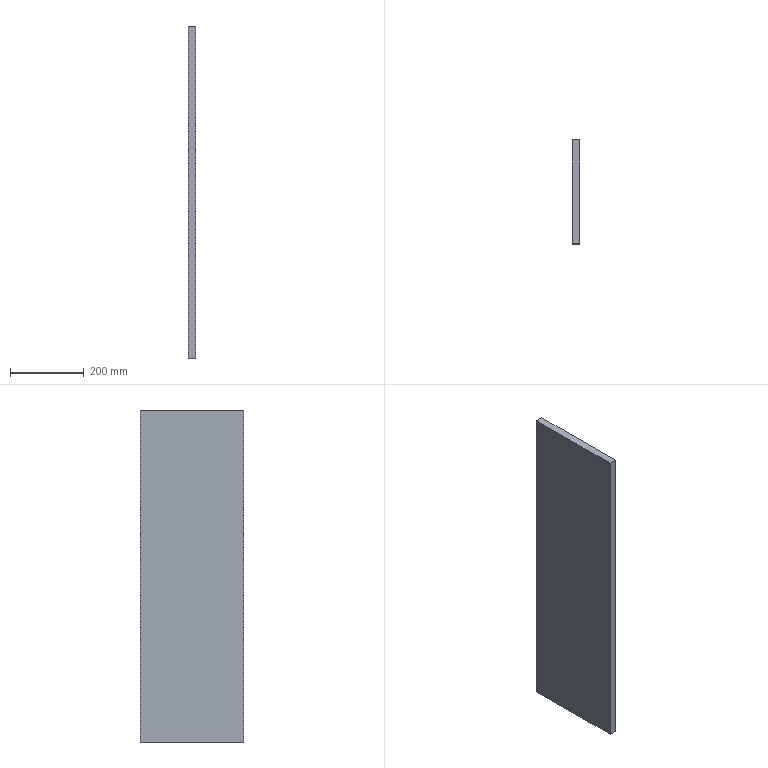Component | SolidWorks | BasePlate-1 | 1 solid | 6 faces | box 20 x 281.2 x 900 mm | volume 5061600 mm3 | plane 6 | material 45
build123d program:
from build123d import *

# Parameters (mm, degrees)
SKETCH1_W           = 900
SKETCH1_H           = 281.2
BOSS_EXTRUDE1_DEPTH = 20


with BuildPart() as part:
    # Sketch1 → Boss-Extrude1 (new body)
    with BuildSketch(Plane.XY):
        Rectangle(SKETCH1_W, SKETCH1_H)
    extrude(amount=BOSS_EXTRUDE1_DEPTH)


solid = part.part

# Placed as in the assembly
solid = solid.moved(Location((-261.359, -192.885, 1152), (0, 90, 0)))
STEP:
#1=CARTESIAN_POINT('',(-9.502,-2.058,27.638));
#2=VERTEX_POINT('',#1);
#3=CARTESIAN_POINT('',(-9.502,-13.129,27.638));
#4=VERTEX_POINT('',#3);
#5=CARTESIAN_POINT('',(-9.502,-13.129,27.638));
#6=DIRECTION('',(0.,-1.,0.));
#7=VECTOR('',#6,39.37);
#8=LINE('',#5,#7);
#9=EDGE_CURVE('',#2,#4,#8,.T.);
#10=ORIENTED_EDGE('',*,*,#9,.T.);
#11=CARTESIAN_POINT('',(-10.29,-13.129,27.638));
#12=VERTEX_POINT('',#11);
#13=CARTESIAN_POINT('',(-10.29,-13.129,27.638));
#14=DIRECTION('',(1.,0.,0.));
#15=VECTOR('',#14,39.37);
#16=LINE('',#13,#15);
#17=EDGE_CURVE('',#12,#4,#16,.T.);
#18=ORIENTED_EDGE('',*,*,#17,.F.);
#19=CARTESIAN_POINT('',(-10.29,-2.058,27.638));
#20=VERTEX_POINT('',#19);
#21=CARTESIAN_POINT('',(-10.29,-13.129,27.638));
#22=DIRECTION('',(0.,-1.,0.));
#23=VECTOR('',#22,39.37);
#24=LINE('',#21,#23);
#25=EDGE_CURVE('',#20,#12,#24,.T.);
#26=ORIENTED_EDGE('',*,*,#25,.F.);
#27=CARTESIAN_POINT('',(-10.29,-2.058,27.638));
#28=DIRECTION('',(1.,0.,0.));
#29=VECTOR('',#28,39.37);
#30=LINE('',#27,#29);
#31=EDGE_CURVE('',#20,#2,#30,.T.);
#32=ORIENTED_EDGE('',*,*,#31,.T.);
#33=EDGE_LOOP('',(#10,#18,#26,#32));
#34=FACE_OUTER_BOUND('',#33,.T.);
#35=CARTESIAN_POINT('',(-10.29,-13.129,27.638));
#36=DIRECTION('',(0.,0.,1.));
#37=DIRECTION('',(1.,0.,0.));
#38=AXIS2_PLACEMENT_3D('',#35,#36,#37);
#39=PLANE('',#38);
#40=ADVANCED_FACE('',(#34),#39,.F.);
#41=CARTESIAN_POINT('',(-9.502,-13.129,63.071));
#42=VERTEX_POINT('',#41);
#43=CARTESIAN_POINT('',(-9.502,-13.129,63.071));
#44=DIRECTION('',(0.,0.,1.));
#45=VECTOR('',#44,39.37);
#46=LINE('',#43,#45);
#47=EDGE_CURVE('',#4,#42,#46,.T.);
#48=ORIENTED_EDGE('',*,*,#47,.T.);
#49=CARTESIAN_POINT('',(-10.29,-13.129,63.071));
#50=VERTEX_POINT('',#49);
#51=CARTESIAN_POINT('',(-10.29,-13.129,63.071));
#52=DIRECTION('',(1.,0.,0.));
#53=VECTOR('',#52,39.37);
#54=LINE('',#51,#53);
#55=EDGE_CURVE('',#50,#42,#54,.T.);
#56=ORIENTED_EDGE('',*,*,#55,.F.);
#57=CARTESIAN_POINT('',(-10.29,-13.129,63.071));
#58=DIRECTION('',(0.,0.,1.));
#59=VECTOR('',#58,39.37);
#60=LINE('',#57,#59);
#61=EDGE_CURVE('',#12,#50,#60,.T.);
#62=ORIENTED_EDGE('',*,*,#61,.F.);
#63=ORIENTED_EDGE('',*,*,#17,.T.);
#64=EDGE_LOOP('',(#48,#56,#62,#63));
#65=FACE_OUTER_BOUND('',#64,.T.);
#66=CARTESIAN_POINT('',(-10.29,-13.129,63.071));
#67=DIRECTION('',(0.,1.,-0.));
#68=DIRECTION('',(0.,-0.,-1.));
#69=AXIS2_PLACEMENT_3D('',#66,#67,#68);
#70=PLANE('',#69);
#71=ADVANCED_FACE('',(#65),#70,.F.);
#72=CARTESIAN_POINT('',(-9.502,-2.058,63.071));
#73=VERTEX_POINT('',#72);
#74=CARTESIAN_POINT('',(-9.502,-13.129,63.071));
#75=DIRECTION('',(0.,1.,0.));
#76=VECTOR('',#75,39.37);
#77=LINE('',#74,#76);
#78=EDGE_CURVE('',#42,#73,#77,.T.);
#79=ORIENTED_EDGE('',*,*,#78,.T.);
#80=CARTESIAN_POINT('',(-10.29,-2.058,63.071));
#81=VERTEX_POINT('',#80);
#82=CARTESIAN_POINT('',(-10.29,-2.058,63.071));
#83=DIRECTION('',(1.,0.,0.));
#84=VECTOR('',#83,39.37);
#85=LINE('',#82,#84);
#86=EDGE_CURVE('',#81,#73,#85,.T.);
#87=ORIENTED_EDGE('',*,*,#86,.F.);
#88=CARTESIAN_POINT('',(-10.29,-13.129,63.071));
#89=DIRECTION('',(0.,1.,0.));
#90=VECTOR('',#89,39.37);
#91=LINE('',#88,#90);
#92=EDGE_CURVE('',#50,#81,#91,.T.);
#93=ORIENTED_EDGE('',*,*,#92,.F.);
#94=ORIENTED_EDGE('',*,*,#55,.T.);
#95=EDGE_LOOP('',(#79,#87,#93,#94));
#96=FACE_OUTER_BOUND('',#95,.T.);
#97=CARTESIAN_POINT('',(-10.29,-13.129,63.071));
#98=DIRECTION('',(0.,0.,-1.));
#99=DIRECTION('',(-1.,0.,0.));
#100=AXIS2_PLACEMENT_3D('',#97,#98,#99);
#101=PLANE('',#100);
#102=ADVANCED_FACE('',(#96),#101,.F.);
#103=CARTESIAN_POINT('',(-9.502,-2.058,63.071));
#104=DIRECTION('',(0.,-0.,-1.));
#105=VECTOR('',#104,39.37);
#106=LINE('',#103,#105);
#107=EDGE_CURVE('',#73,#2,#106,.T.);
#108=ORIENTED_EDGE('',*,*,#107,.T.);
#109=ORIENTED_EDGE('',*,*,#31,.F.);
#110=CARTESIAN_POINT('',(-10.29,-2.058,63.071));
#111=DIRECTION('',(0.,-0.,-1.));
#112=VECTOR('',#111,39.37);
#113=LINE('',#110,#112);
#114=EDGE_CURVE('',#81,#20,#113,.T.);
#115=ORIENTED_EDGE('',*,*,#114,.F.);
#116=ORIENTED_EDGE('',*,*,#86,.T.);
#117=EDGE_LOOP('',(#108,#109,#115,#116));
#118=FACE_OUTER_BOUND('',#117,.T.);
#119=CARTESIAN_POINT('',(-10.29,-2.058,63.071));
#120=DIRECTION('',(0.,-1.,0.));
#121=DIRECTION('',(0.,0.,1.));
#122=AXIS2_PLACEMENT_3D('',#119,#120,#121);
#123=PLANE('',#122);
#124=ADVANCED_FACE('',(#118),#123,.F.);
#125=ORIENTED_EDGE('',*,*,#25,.T.);
#126=ORIENTED_EDGE('',*,*,#61,.T.);
#127=ORIENTED_EDGE('',*,*,#92,.T.);
#128=ORIENTED_EDGE('',*,*,#114,.T.);
#129=EDGE_LOOP('',(#125,#126,#127,#128));
#130=FACE_OUTER_BOUND('',#129,.T.);
#131=CARTESIAN_POINT('',(-10.29,-7.594,45.354));
#132=DIRECTION('',(-1.,0.,0.));
#133=DIRECTION('',(0.,0.,1.));
#134=AXIS2_PLACEMENT_3D('',#131,#132,#133);
#135=PLANE('',#134);
#136=ADVANCED_FACE('',(#130),#135,.T.);
#137=ORIENTED_EDGE('',*,*,#9,.F.);
#138=ORIENTED_EDGE('',*,*,#107,.F.);
#139=ORIENTED_EDGE('',*,*,#78,.F.);
#140=ORIENTED_EDGE('',*,*,#47,.F.);
#141=EDGE_LOOP('',(#137,#138,#139,#140));
#142=FACE_OUTER_BOUND('',#141,.T.);
#143=CARTESIAN_POINT('',(-9.502,-7.594,45.354));
#144=DIRECTION('',(-1.,0.,0.));
#145=DIRECTION('',(0.,0.,1.));
#146=AXIS2_PLACEMENT_3D('',#143,#144,#145);
#147=PLANE('',#146);
#148=ADVANCED_FACE('',(#142),#147,.F.);
#149=CLOSED_SHELL('',(#40,#71,#102,#124,#136,#148));
#150=MANIFOLD_SOLID_BREP('',#149);
#151=CARTESIAN_POINT('',(0.,0.,0.));
#152=DIRECTION('',(0.,0.,1.));
#153=DIRECTION('',(1.,0.,0.));
#154=AXIS2_PLACEMENT_3D('',#151,#152,#153);
#155=(LENGTH_UNIT()NAMED_UNIT(*)SI_UNIT($,.METRE.));
#156=LENGTH_MEASURE_WITH_UNIT(LENGTH_MEASURE(0.0254),#155);
#157=DIMENSIONAL_EXPONENTS(1.,0.,0.,0.,0.,0.,0.);
#158=(CONVERSION_BASED_UNIT('',#156)LENGTH_UNIT()NAMED_UNIT(#157));
#159=UNCERTAINTY_MEASURE_WITH_UNIT(LENGTH_MEASURE(0.00001),#158,'','');
#160=(NAMED_UNIT(*)PLANE_ANGLE_UNIT()SI_UNIT($,.RADIAN.));
#161=(NAMED_UNIT(*)SI_UNIT($,.STERADIAN.)SOLID_ANGLE_UNIT());
#162=(GEOMETRIC_REPRESENTATION_CONTEXT(3)GLOBAL_UNCERTAINTY_ASSIGNED_CONTEXT((#159))GLOBAL_UNIT_ASSIGNED_CONTEXT((#158,#160,#161))REPRESENTATION_CONTEXT('',''));
#163=ADVANCED_BREP_SHAPE_REPRESENTATION('',(#150,#154),#162);
#164=COLOUR_RGB('',0.7922,0.8196,0.9333);
#165=FILL_AREA_STYLE_COLOUR('',#164);
#166=FILL_AREA_STYLE('',(#165));
#167=SURFACE_STYLE_FILL_AREA(#166);
#168=SURFACE_SIDE_STYLE('',(#167));
#169=SURFACE_STYLE_USAGE(.BOTH.,#168);
#170=PRESENTATION_STYLE_ASSIGNMENT((#169));
#171=STYLED_ITEM('',(#170),#150);
#172=PRESENTATION_LAYER_ASSIGNMENT('','',(#171));
#173=(LENGTH_UNIT()NAMED_UNIT(*)SI_UNIT($,.METRE.));
#174=LENGTH_MEASURE_WITH_UNIT(LENGTH_MEASURE(0.0254),#173);
#175=DIMENSIONAL_EXPONENTS(1.,0.,0.,0.,0.,0.,0.);
#176=(CONVERSION_BASED_UNIT('',#174)LENGTH_UNIT()NAMED_UNIT(#175));
#177=UNCERTAINTY_MEASURE_WITH_UNIT(LENGTH_MEASURE(0.00001),#176,'','');
#178=(NAMED_UNIT(*)PLANE_ANGLE_UNIT()SI_UNIT($,.RADIAN.));
#179=(NAMED_UNIT(*)SI_UNIT($,.STERADIAN.)SOLID_ANGLE_UNIT());
#180=(GEOMETRIC_REPRESENTATION_CONTEXT(3)GLOBAL_UNCERTAINTY_ASSIGNED_CONTEXT((#177))GLOBAL_UNIT_ASSIGNED_CONTEXT((#176,#178,#179))REPRESENTATION_CONTEXT('',''));
#181=MECHANICAL_DESIGN_GEOMETRIC_PRESENTATION_REPRESENTATION('',(#171),#180);